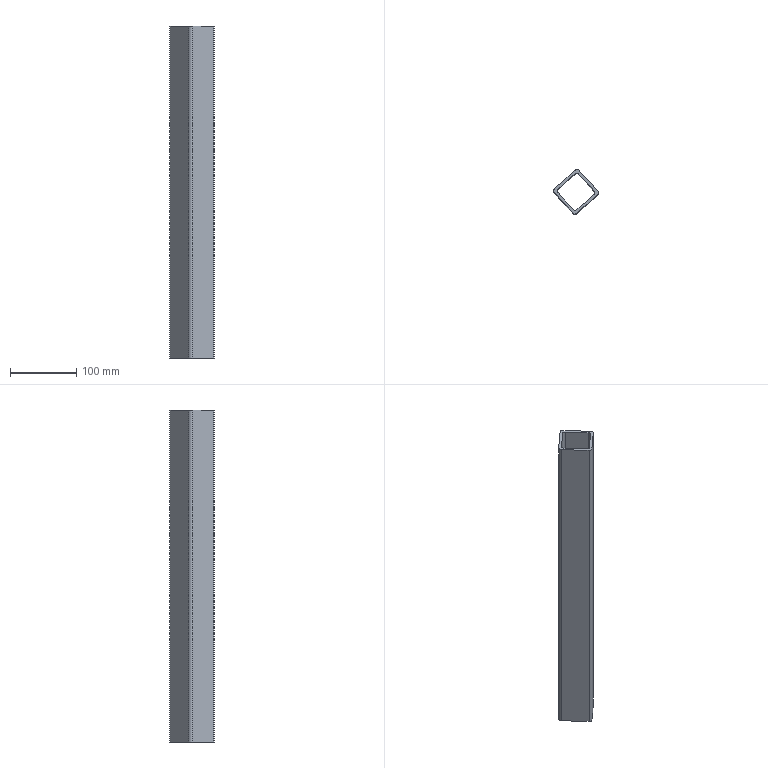Component | NX | ADJ_BRKT_TOP_BEAM | 1 solid | 18 faces | volume 368000 mm3 | plane 10 | cylinder 8 | commonest cylinder face diameters 8 x8